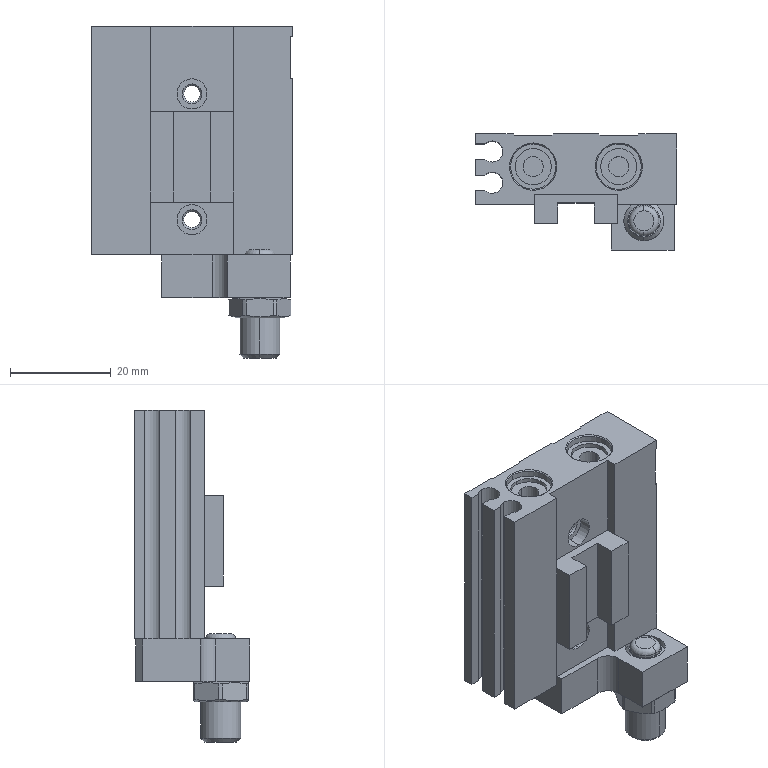Component | SolidWorks | SL010-LeftStreamline-1-1_SL010-SideClampAssembly-DB-1-1_SL010-HLQ8X10SAF(0)+(DS1-H-2)-DB-1-1_SL010-HLQ8X10-S-AF-0-H-2-body-DB-1-1 | 1 solid | 280 faces | box 40 x 23 x 66 mm | volume 23770 mm3 | cylinder 102 | plane 100 | cone 66 | torus 12 | commonest cylinder face diameters 2.459 x12 8 x8 2.5 x8 5 x8 5.5 x8 9 x8 3 x7 6 x7
build123d program:
from build123d import *

# Parameters (mm, degrees)
BOSS_EXTRUDE1_DEPTH  = 45.5
BOSS_EXTRUDE2_DEPTH  = 18
SKETCH9_W            = 8.5
SKETCH9_H            = 0.5
CUT_EXTRUDE1_DEPTH   = 14
LPATTERN1_COUNT      = 2
LPATTERN1_PITCH      = 15
LPATTERN1_COUNT_DIR2 = 2
LPATTERN1_PITCH_DIR2 = 6.5
BOSS_EXTRUDE3_DEPTH  = 8.5
LPATTERN2_COUNT      = 2
LPATTERN2_PITCH      = 15
LPATTERN2_COUNT_DIR2 = 2
LPATTERN2_PITCH_DIR2 = 6.5
SKETCH19_W           = 8.5
SKETCH19_H           = 4
SKETCH21_R           = 7
CUT_EXTRUDE2_DEPTH   = 4
SKETCH22_R           = 1.5
CUT_EXTRUDE3_DEPTH   = 3
CUT_EXTRUDE4_DEPTH   = 3


with BuildPart() as part:
    # Sketch1 → Boss-Extrude1 (new body)
    with BuildSketch(Plane(origin=(0, 0, 0), x_dir=(0, 0, -1), z_dir=(1, 0, 0))):
        with BuildLine():
            Line((-7.5, -8.2), (-7.5, -20))
            Line((-7.5, -20), (-4.7, -20))
            Line((-4.7, -20), (-4.7, -18.12))
            ThreePointArc((-4.7, -18.12), (-3.2, -14.55), (-1.7, -18.12))
            Line((-1.7, -18.12), (-1.7, -20))
            Line((-1.7, -20), (1.5, -20))
            Line((1.5, -20), (1.5, -18.12))
            ThreePointArc((1.5, -18.12), (3, -14.55), (4.5, -18.12))
            Line((4.5, -18.12), (4.5, -20))
            Line((4.5, -20), (6.5, -20))
            Line((6.5, -20), (6.5, -12.5))
            Line((6.5, -12.5), (6.2, -12.2))
            Line((6.2, -12.2), (6.2, -4.8))
            Line((6.2, -4.8), (6.5, -4.5))
            Line((6.5, -4.5), (6.5, 4.5))
            Line((6.5, 4.5), (6.2, 4.8))
            Line((6.2, 4.8), (6.2, 12.2))
            Line((6.2, 12.2), (6.5, 12.5))
            Line((6.5, 12.5), (6.5, 20))
            Line((6.5, 20), (-7.5, 20))
            Line((-7.5, 20), (-7.5, 8.2))
            Line((-7.5, 8.2), (-5.5, 8.2))
            Line((-5.5, 8.2), (-5.5, -8.2))
            Line((-5.5, -8.2), (-7.5, -8.2))
        make_face()
    extrude(amount=BOSS_EXTRUDE1_DEPTH)

    # Sketch2 → Cut-Revolve1 (revolve, cut)
    with BuildSketch(Plane.XY, mode=Mode.PRIVATE) as cut_revolve1_sk:
        Polygon((0, 8.5), (0, 13.212), (0.2121, 13), (1.4, 13), (1.4, 12.1), (2.2, 12.1), (2.2, 10.5), (15, 10.5), (15, 12.5), (39.7, 12.5), (39.7, 8.5), align=None)
    revolve(cut_revolve1_sk.sketch.rotate(Axis((39.7, 8.5, 0), (-1, 0, 0)), 180), axis=Axis((39.7, 8.5, 0), (-1, 0, 0)), mode=Mode.SUBTRACT)

    # Sketch3 → Cut-Revolve2 (revolve, cut)
    with BuildSketch(Plane.XY, mode=Mode.PRIVATE) as cut_revolve2_sk:
        Polygon((0, -8.5), (0, -3.788), (0.2121, -4), (1.4, -4), (1.4, -4.9), (2.2, -4.9), (2.2, -6.5), (15, -6.5), (15, -4.5), (39.7, -4.5), (39.7, -8.5), align=None)
    revolve(cut_revolve2_sk.sketch.rotate(Axis((39.7, -8.5, 0), (-1, 0, 0)), 270), axis=Axis((39.7, -8.5, 0), (-1, 0, 0)), mode=Mode.SUBTRACT)

    # Sketch4 → Cut-Revolve3 (revolve, cut)
    with BuildSketch(Plane.XY, mode=Mode.PRIVATE) as cut_revolve3_sk:
        Polygon((43.2, -8.5), (43.2, -5.09), (44, -5.09), (44, -4), (45.288, -4), (45.5, -3.788), (45.5, -8.5), align=None)
    revolve(cut_revolve3_sk.sketch.rotate(Axis((45.5, -8.5, 0), (-1, 0, 0)), 270), axis=Axis((45.5, -8.5, 0), (-1, 0, 0)), mode=Mode.SUBTRACT)

    # Sketch5 → Cut-Revolve4 (revolve, cut)
    with BuildSketch(Plane.XY, mode=Mode.PRIVATE) as cut_revolve4_sk:
        Polygon((43.2, 8.5), (43.2, 11.91), (44, 11.91), (44, 13), (45.288, 13), (45.5, 13.212), (45.5, 8.5), align=None)
    revolve(cut_revolve4_sk.sketch.rotate(Axis((45.5, 8.5, 0), (-1, 0, 0)), 180), axis=Axis((45.5, 8.5, 0), (-1, 0, 0)), mode=Mode.SUBTRACT)

    # Sketch6 → Boss-Extrude2 (add)
    with BuildSketch(Plane(origin=(17, 0, 0), x_dir=(0, 0, -1), z_dir=(1, 0, 0))):
        Polygon((-11.2, 3.6), (-7.2, 3.6), (-7.2, -3.6), (-11.2, -3.6), (-11.2, -8.2), (-5.5, -8.2), (-5.5, 8.2), (-11.2, 8.2), align=None)
    extrude(amount=BOSS_EXTRUDE2_DEPTH)

    # Sketch7 → Cut-Revolve5 (revolve, cut)
    with BuildSketch(Plane.XY, mode=Mode.PRIVATE) as cut_revolve5_sk:
        Polygon((35.5, 11), (34.9, 11), (34.9, 14), (33.433, 14), (33.433, 19.567), (33, 20), (35.5, 20), align=None)
    revolve(cut_revolve5_sk.sketch.rotate(Axis((35.5, 20, 0), (0, -1, 0)), 90), axis=Axis((35.5, 20, 0), (0, -1, 0)), mode=Mode.SUBTRACT)

    # Sketch8 → Cut-Revolve6 (revolve, cut)
    with BuildSketch(Plane.XY, mode=Mode.PRIVATE) as cut_revolve6_sk:
        Polygon((17.5, 11), (16.9, 11), (16.9, 14), (15.433, 14), (15.433, 19.567), (15, 20), (17.5, 20), align=None)
    revolve(cut_revolve6_sk.sketch.rotate(Axis((17.5, 20, 0), (0, -1, 0)), 90), axis=Axis((17.5, 20, 0), (0, -1, 0)), mode=Mode.SUBTRACT)

    # Sketch9 → Cut-Extrude1 (cut)
    with BuildSketch(Plane.XY.offset(-6.5)):
        with Locations((6.25, 19.75)):
            Rectangle(SKETCH9_W, SKETCH9_H)
    extrude(amount=CUT_EXTRUDE1_DEPTH, mode=Mode.SUBTRACT)

    # Sketch10 → Cut-Revolve7 (revolve, cut)
    with BuildSketch(Plane(origin=(6.2, 0, 0), x_dir=(0, 0, -1), z_dir=(1, 0, 0)), mode=Mode.PRIVATE) as cut_revolve7_sk:
        Polygon((2.5, 15), (1.27, 15), (1.27, 19.23), (1, 19.5), (2.5, 19.5), align=None)
    revolve(cut_revolve7_sk.sketch.rotate(Axis((6.2, 19.5, -2.5), (0, -1, 0)), 180), axis=Axis((6.2, 19.5, -2.5), (0, -1, 0)), mode=Mode.SUBTRACT)

    # Sketch11 → Cut-Revolve8 (revolve, cut)
    with BuildSketch(Plane(origin=(6.2, 0, 0), x_dir=(0, 0, -1), z_dir=(1, 0, 0)), mode=Mode.PRIVATE) as cut_revolve8_sk:
        Polygon((-4, 15), (-5.229, 15), (-5.229, 19.23), (-5.5, 19.5), (-4, 19.5), align=None)
    revolve(cut_revolve8_sk.sketch.rotate(Axis((6.2, 19.5, 4), (0, -1, 0)), 180), axis=Axis((6.2, 19.5, 4), (0, -1, 0)), mode=Mode.SUBTRACT)

    # Sketch12 → Cut-Revolve9 (revolve, cut)
    with BuildSketch(Plane(origin=(0, 0, 0), x_dir=(1, 0, 0), z_dir=(0, 1, 0)), mode=Mode.PRIVATE) as cut_revolve9_sk:
        Polygon((13.5, -6.5), (10.146, -6.5), (10.5, -6.146), (10.5, -3.1), (11.525, -3.1), (11.879, -2.746), (11.879, 6.121), (11.5, 6.5), (13.5, 6.5), align=None)
    revolve(cut_revolve9_sk.sketch.rotate(Axis((13.5, 0, -6.5), (0, 0, 1)), 180), axis=Axis((13.5, 0, -6.5), (0, 0, 1)), mode=Mode.SUBTRACT)

    # Sketch13 → Cut-Revolve10 (revolve, cut)
    with BuildSketch(Plane(origin=(0, 0, 0), x_dir=(1, 0, 0), z_dir=(0, 1, 0)), mode=Mode.PRIVATE) as cut_revolve10_sk:
        Polygon((38.5, -6.5), (35.146, -6.5), (35.5, -6.146), (35.5, -3.1), (36.525, -3.1), (36.879, -2.746), (36.879, 6.121), (36.5, 6.5), (38.5, 6.5), align=None)
    revolve(cut_revolve10_sk.sketch.rotate(Axis((38.5, 0, -6.5), (0, 0, 1)), 180), axis=Axis((38.5, 0, -6.5), (0, 0, 1)), mode=Mode.SUBTRACT)

    # Sketch14 → Cut-Revolve11 (revolve, cut)
    with BuildSketch(Plane(origin=(0, 0, 0), x_dir=(1, 0, 0), z_dir=(0, 1, 0)), mode=Mode.PRIVATE) as cut_revolve11_sk:
        Polygon((41.29, 3), (42, 4.229), (45.23, 4.229), (45.5, 4.5), (45.5, 3), align=None)
    cut_revolve11 = revolve(cut_revolve11_sk.sketch.rotate(Axis((45.5, 0, -3), (-1, 0, 0)), 180), axis=Axis((45.5, 0, -3), (-1, 0, 0)), mode=Mode.SUBTRACT)

    # LPattern1: Cut-Revolve11 2 × 2
    with Locations(*[(0, i * LPATTERN1_PITCH, j * LPATTERN1_PITCH_DIR2) for i in range(LPATTERN1_COUNT) for j in range(LPATTERN1_COUNT_DIR2) if (i, j) != (0, 0)]):
        add(cut_revolve11, mode=Mode.SUBTRACT)

    # Sketch16 → Boss-Extrude3 (add)
    with BuildSketch(Plane(origin=(45.5, 0, 0), x_dir=(0, 0, -1), z_dir=(1, 0, 0))):
        with BuildLine():
            Line((-16.5, 7), (-9.77, 7))
            ThreePointArc((-9.77, 7), (-7.649, 6.121), (-6.77, 4))
            Line((-6.77, 4), (-6.77, -6))
            Line((-6.77, -6), (4.78, -6))
            Line((4.78, -6), (6.23, -4.55))
            Line((6.23, -4.55), (6.23, 18.05))
            Line((6.23, 18.05), (4.78, 19.5))
            Line((4.78, 19.5), (-16.5, 19.5))
            Line((-16.5, 19.5), (-16.5, 7))
        make_face()
    extrude(amount=BOSS_EXTRUDE3_DEPTH)

    # Sketch17 → Cut-Revolve12 (revolve, cut)
    with BuildSketch(Plane(origin=(0, 0, 0), x_dir=(1, 0, 0), z_dir=(0, 1, 0)), mode=Mode.PRIVATE) as cut_revolve12_sk:
        with BuildLine():
            Line((50.765, 3), (51.487, 4.25))
            Line((51.487, 4.25), (53.4, 4.25))
            Line((53.4, 4.25), (53.4, 5.2))
            ThreePointArc((53.4, 5.2), (53.312, 5.412), (53.1, 5.5))
            Line((53.1, 5.5), (49.4, 5.5))
            Line((49.4, 5.5), (49.4, 5.75))
            Line((49.4, 5.75), (53.788, 5.75))
            Line((53.788, 5.75), (54, 5.962))
            Line((54, 5.962), (54, 3))
            Line((54, 3), (50.765, 3))
        make_face()
    cut_revolve12 = revolve(cut_revolve12_sk.sketch.rotate(Axis((54, 0, -3), (-1, 0, 0)), 180), axis=Axis((54, 0, -3), (-1, 0, 0)), mode=Mode.SUBTRACT)

    # LPattern2: Cut-Revolve12 2 × 2
    with Locations(*[(0, i * LPATTERN2_PITCH, j * LPATTERN2_PITCH_DIR2) for i in range(LPATTERN2_COUNT) for j in range(LPATTERN2_COUNT_DIR2) if (i, j) != (0, 0)]):
        add(cut_revolve12, mode=Mode.SUBTRACT)

    # Sketch19 → Cut-Revolve13 (revolve, cut)
    with BuildSketch(Plane(origin=(0, 13.5, 0), x_dir=(1, 0, 0), z_dir=(0, 1, 0)), mode=Mode.PRIVATE) as cut_revolve13_sk:
        with Locations((49.75, -8.7)):
            Rectangle(SKETCH19_W, SKETCH19_H)
    revolve(cut_revolve13_sk.sketch.rotate(Axis((54, 13.5, 10.7), (-1, 0, 0)), 180), axis=Axis((54, 13.5, 10.7), (-1, 0, 0)), mode=Mode.SUBTRACT)

    # Sketch20 → Revolve1 (revolve)
    with BuildSketch(Plane(origin=(0, 13.5, 0), x_dir=(1, 0, 0), z_dir=(0, 1, 0)), mode=Mode.PRIVATE) as revolve1_sk:
        with BuildLine():
            Line((44.5, -10.7), (44.5, -8.7))
            ThreePointArc((44.5, -8.7), (44.793, -7.993), (45.5, -7.7))
            Line((45.5, -7.7), (46, -7.7))
            Line((46, -7.7), (46, -7.467))
            Line((46, -7.467), (46.767, -6.7))
            Line((46.767, -6.7), (54, -6.7))
            Line((54, -6.7), (54, -5.8))
            Line((54, -5.8), (54.455, -4.55))
            Line((54.455, -4.55), (57.545, -4.55))
            Line((57.545, -4.55), (58, -5.8))
            Line((58, -5.8), (58, -6.7))
            Line((58, -6.7), (65.233, -6.7))
            Line((65.233, -6.7), (66, -7.467))
            Line((66, -7.467), (66, -8.7))
            ThreePointArc((66, -8.7), (65.854, -9.054), (65.5, -9.2))
            Line((65.5, -9.2), (64, -9.2))
            Line((64, -9.2), (63.134, -10.7))
            Line((63.134, -10.7), (44.5, -10.7))
        make_face()
    revolve(revolve1_sk.sketch.rotate(Axis((66, 13.5, 10.7), (-1, 0, 0)), 180), axis=Axis((66, 13.5, 10.7), (-1, 0, 0)))

    # Sketch21 → Cut-Extrude2 (cut)
    with BuildSketch(Plane(origin=(54, 0, 0), x_dir=(0, 0, -1), z_dir=(1, 0, 0))):
        with Locations((-10.7, 13.5)):
            Circle(SKETCH21_R)
        Polygon((-16.2, 10.325), (-10.7, 7.149), (-5.2, 10.325), (-5.2, 16.675), (-10.7, 19.851), (-16.2, 16.675), align=None, mode=Mode.SUBTRACT)
    extrude(amount=CUT_EXTRUDE2_DEPTH, mode=Mode.SUBTRACT)

    # Sketch22 → Cut-Extrude3 (cut)
    with BuildSketch(Plane.XY.offset(-6.5)):
        with Locations(Location((13.5, 14, 0), (0, 0, 270))):
            Circle(SKETCH22_R)
    extrude(amount=CUT_EXTRUDE3_DEPTH, mode=Mode.SUBTRACT)

    # Sketch23 → Cut-Extrude4 (cut)
    with BuildSketch(Plane.XY.offset(-6.5)):
        with BuildLine():
            Line((32, 12.5), (33, 12.5))
            ThreePointArc((33, 12.5), (34.5, 14), (33, 15.5))
            Line((33, 15.5), (32, 15.5))
            ThreePointArc((32, 15.5), (30.5, 14), (32, 12.5))
        make_face()
    extrude(amount=CUT_EXTRUDE4_DEPTH, mode=Mode.SUBTRACT)


solid = part.part

# Placed as in the assembly
solid = solid.moved(Location((-633.5, -115.904, -675.535), (90, 0, -90)))